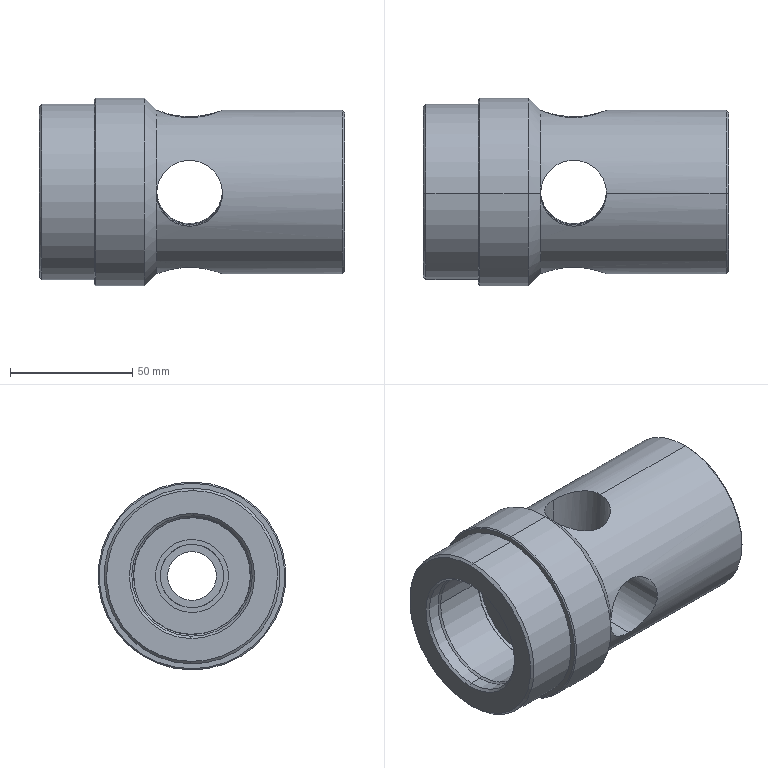Component | SolidWorks | 216InnerTubeAssembly-1_HangingJoint-1 | 1 solid | 55 faces | volume 300831 mm3 | cylinder 32 | cone 14 | plane 9 | commonest cylinder face diameters 27 x8 26 x4 36.01 x2 48.01 x2 49.356 x2 72 x2 77 x2 20 x2 | material Alloy Steel